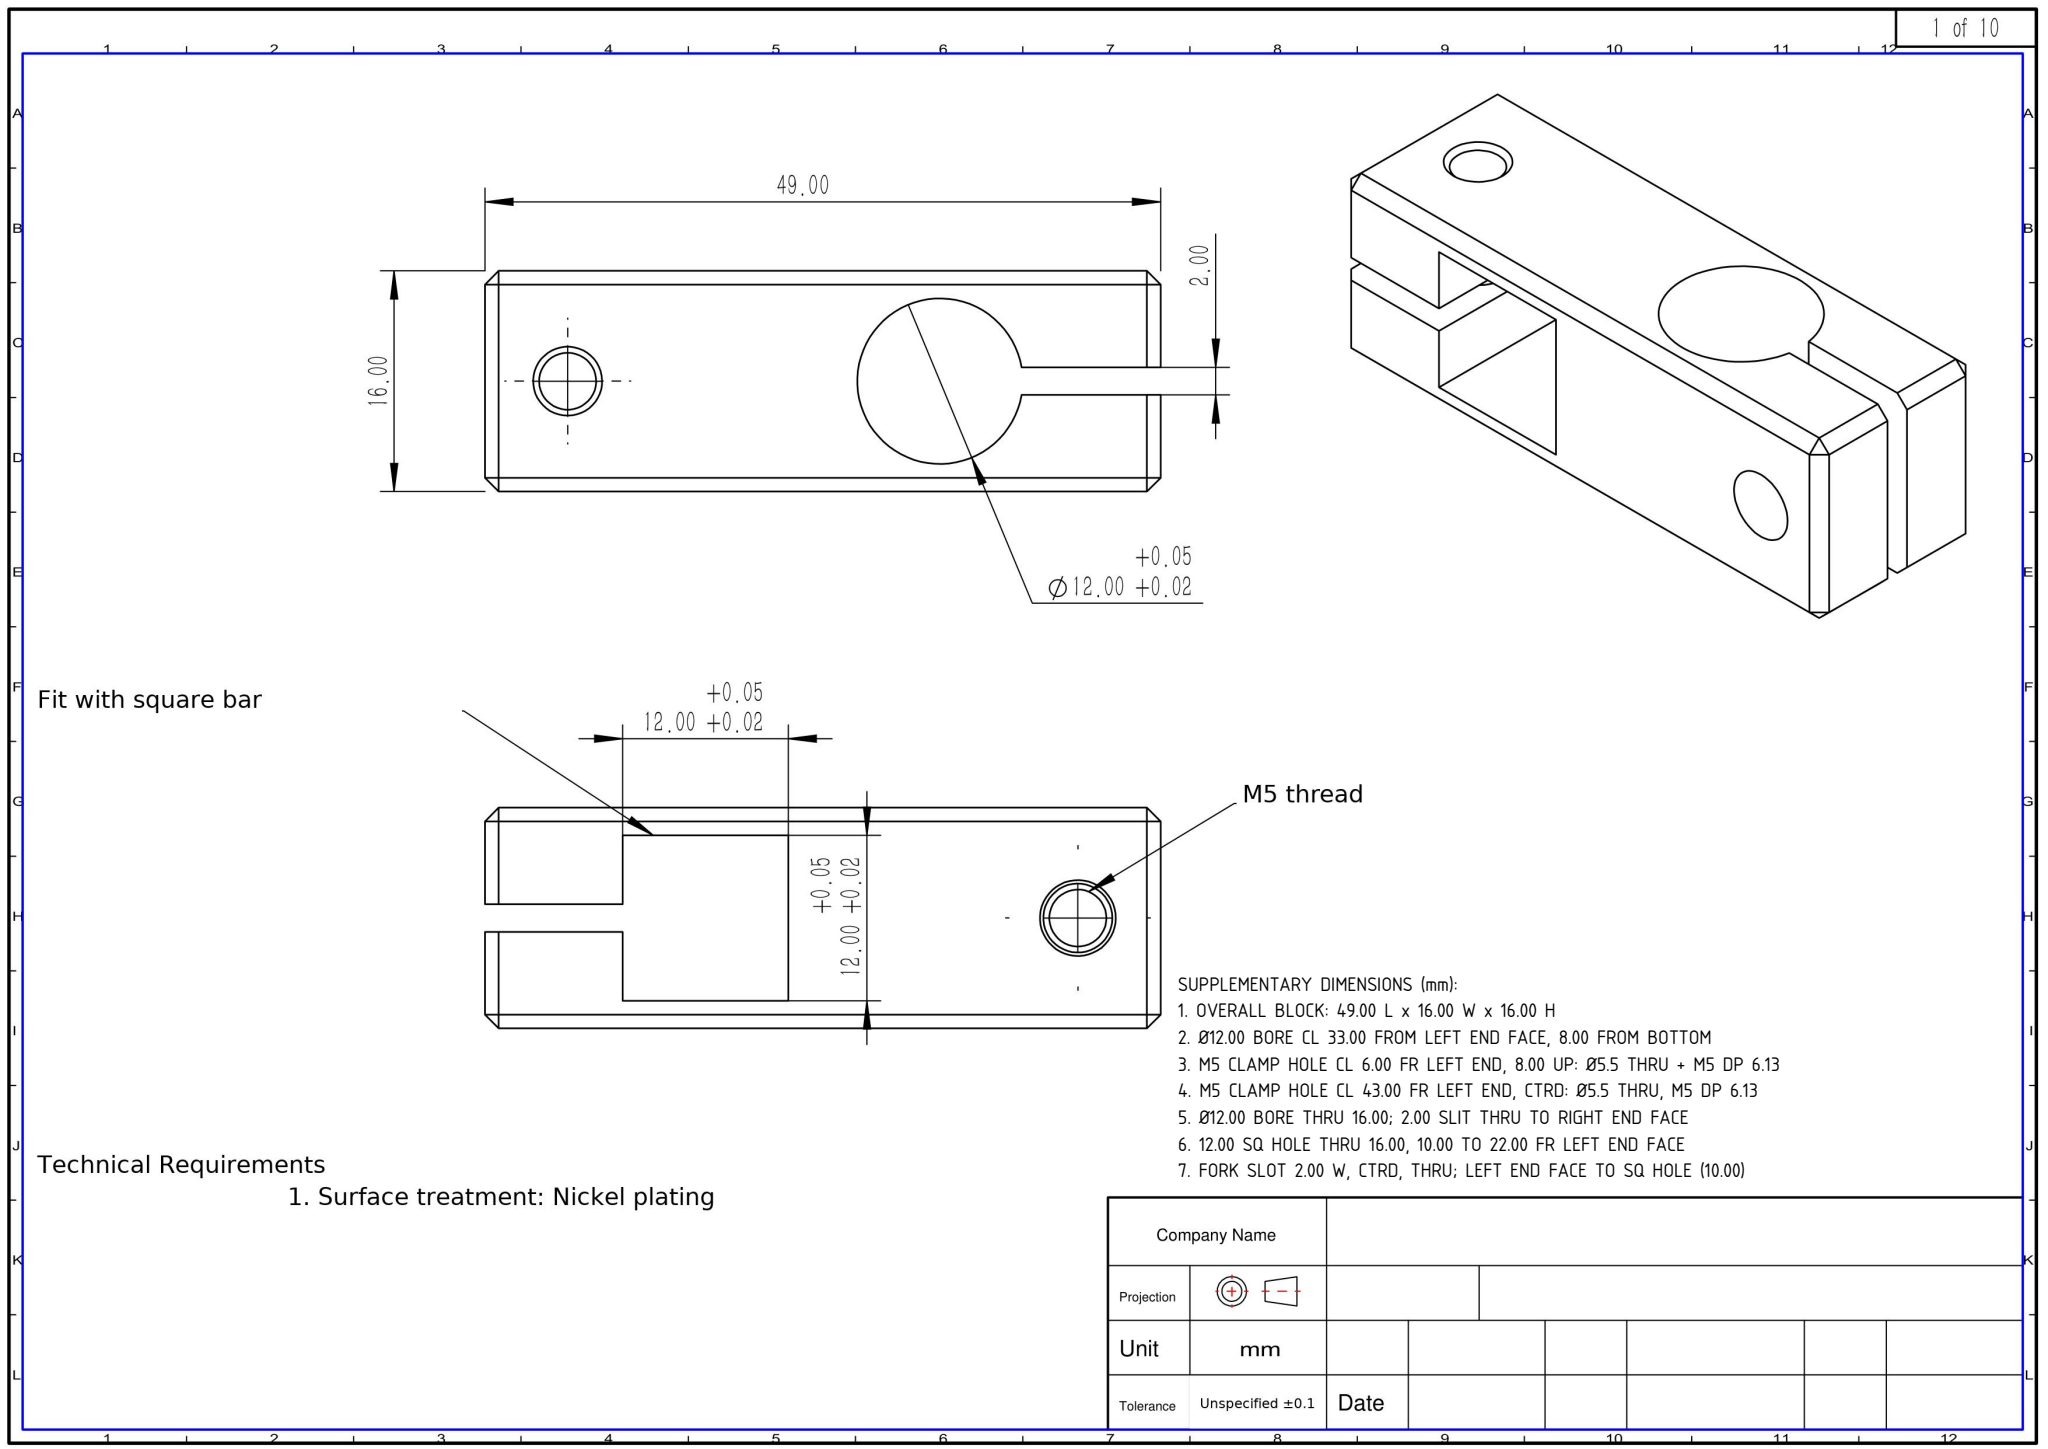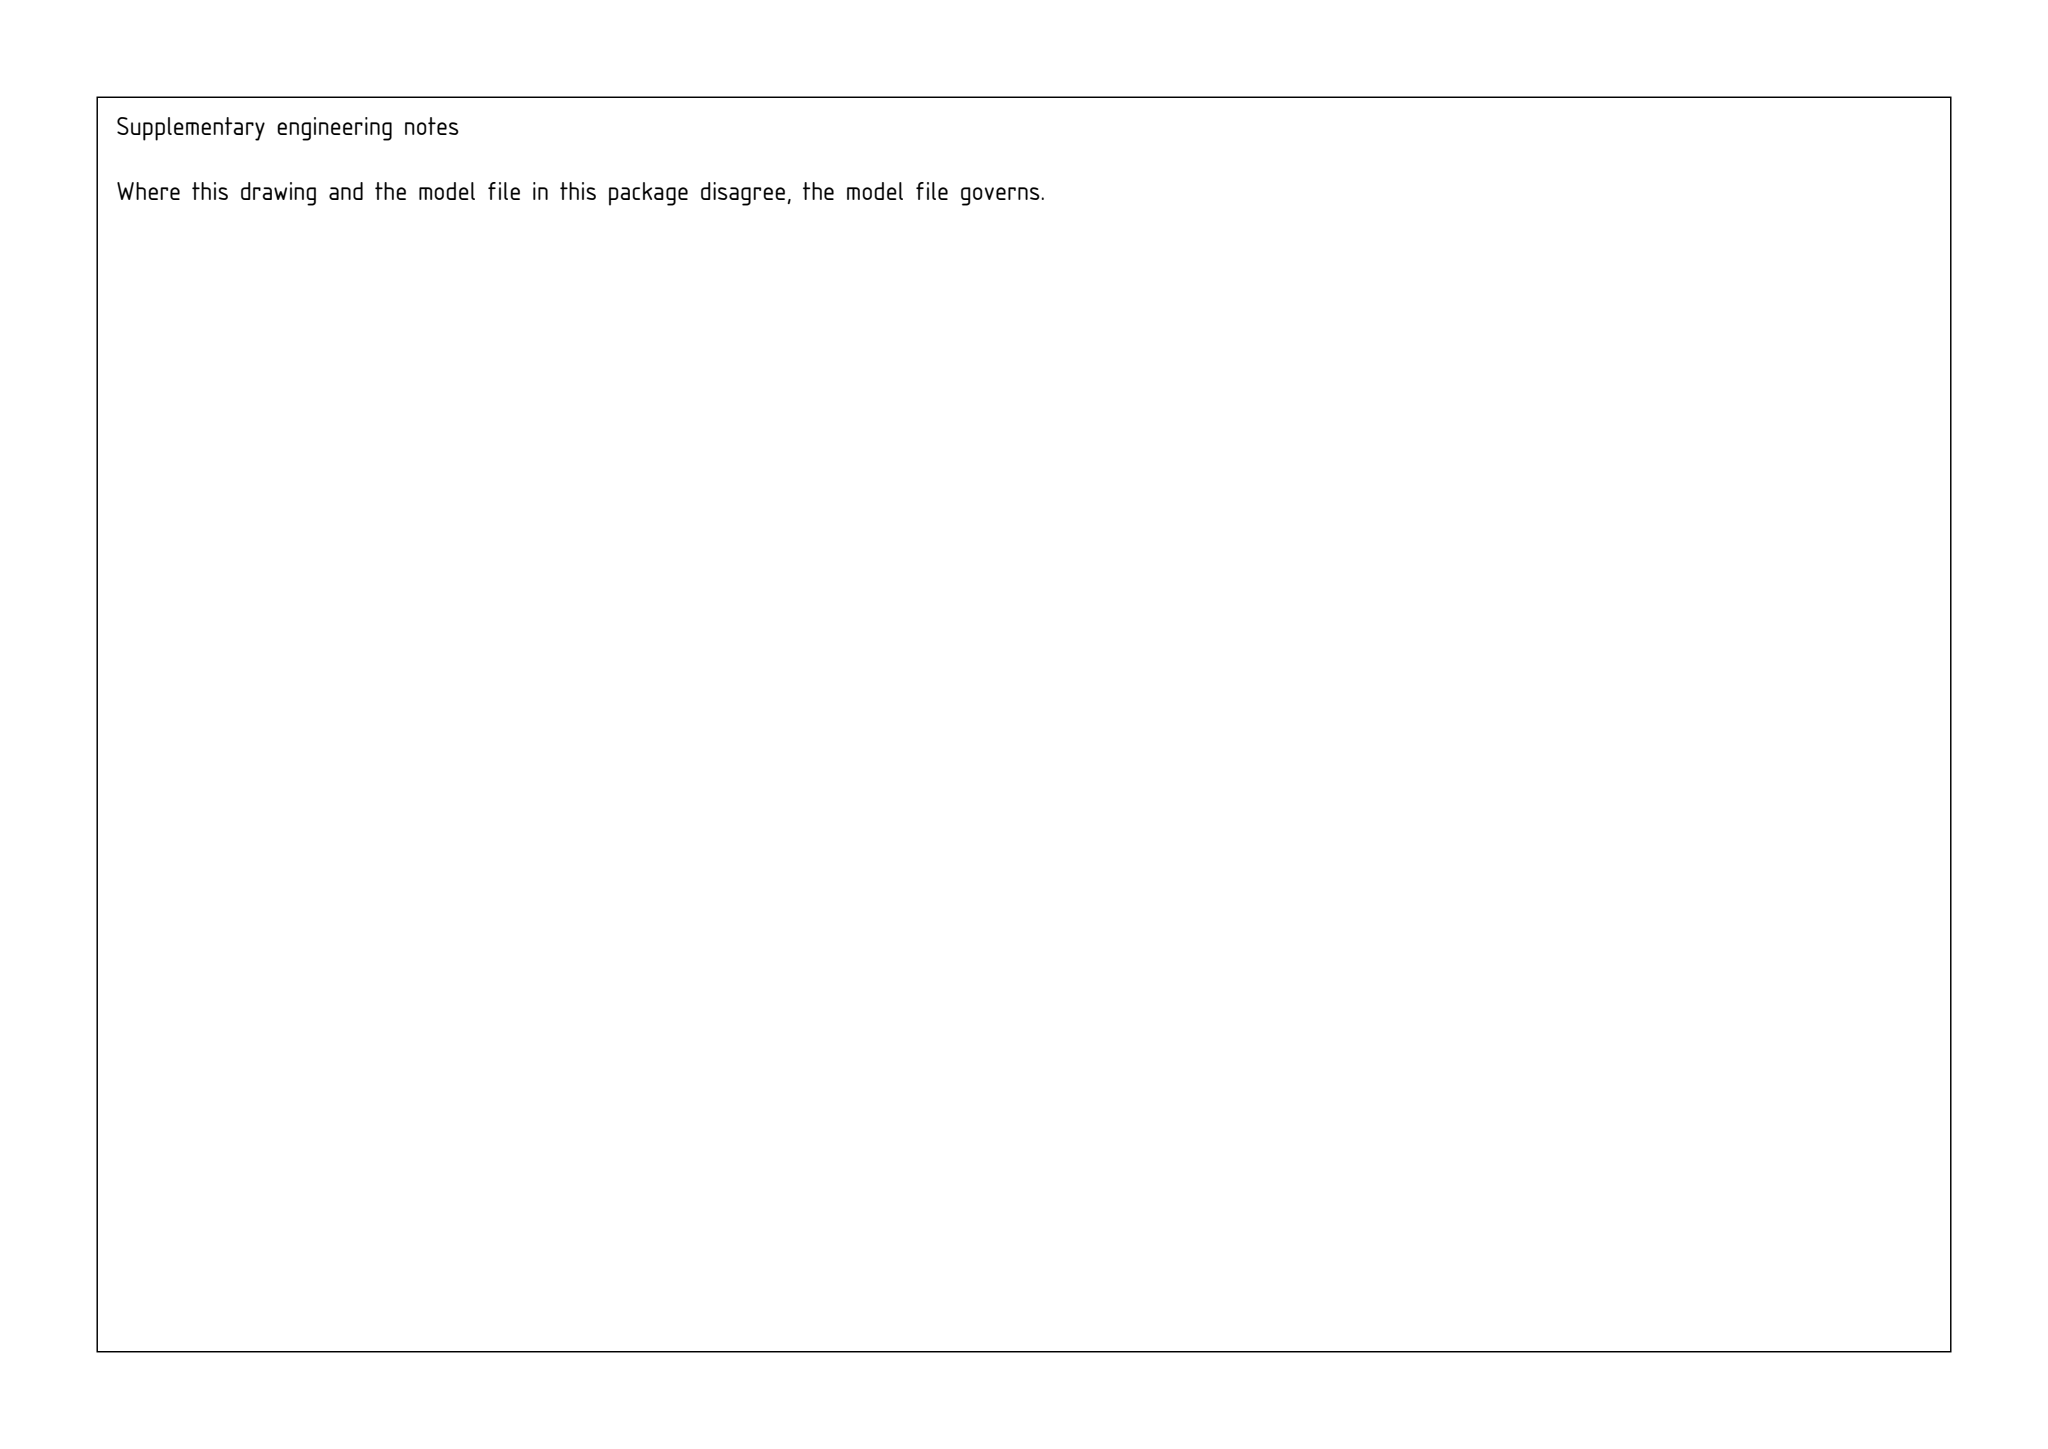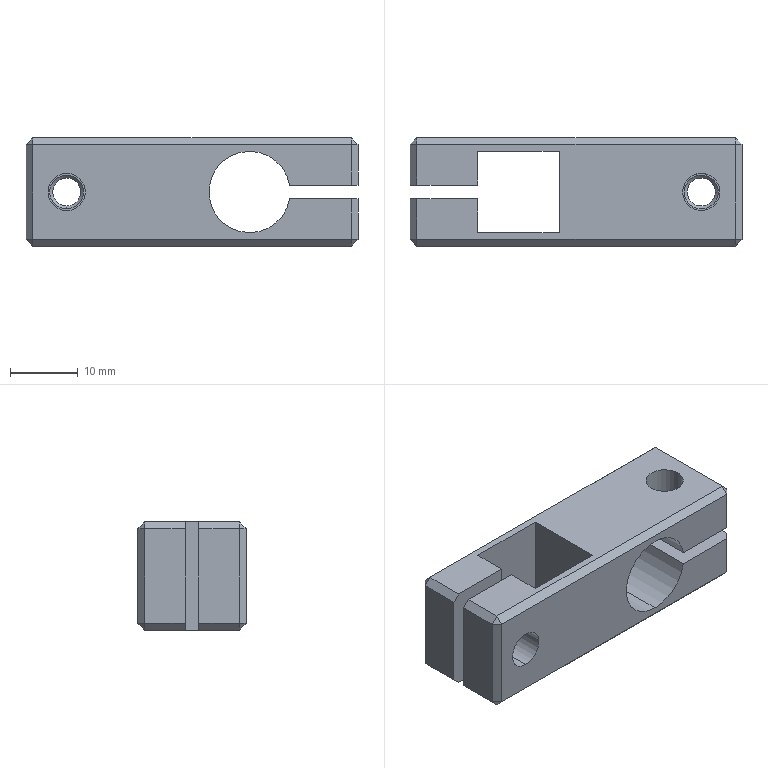Part | SolidWorks | mm | 1 solid | 60 faces | box 49 x 16 x 16 mm | volume 7111 mm3 | plane 41 | cylinder 11 | cone 8 | commonest cylinder face diameters 5.5 x4 4.134 x4 12 x3